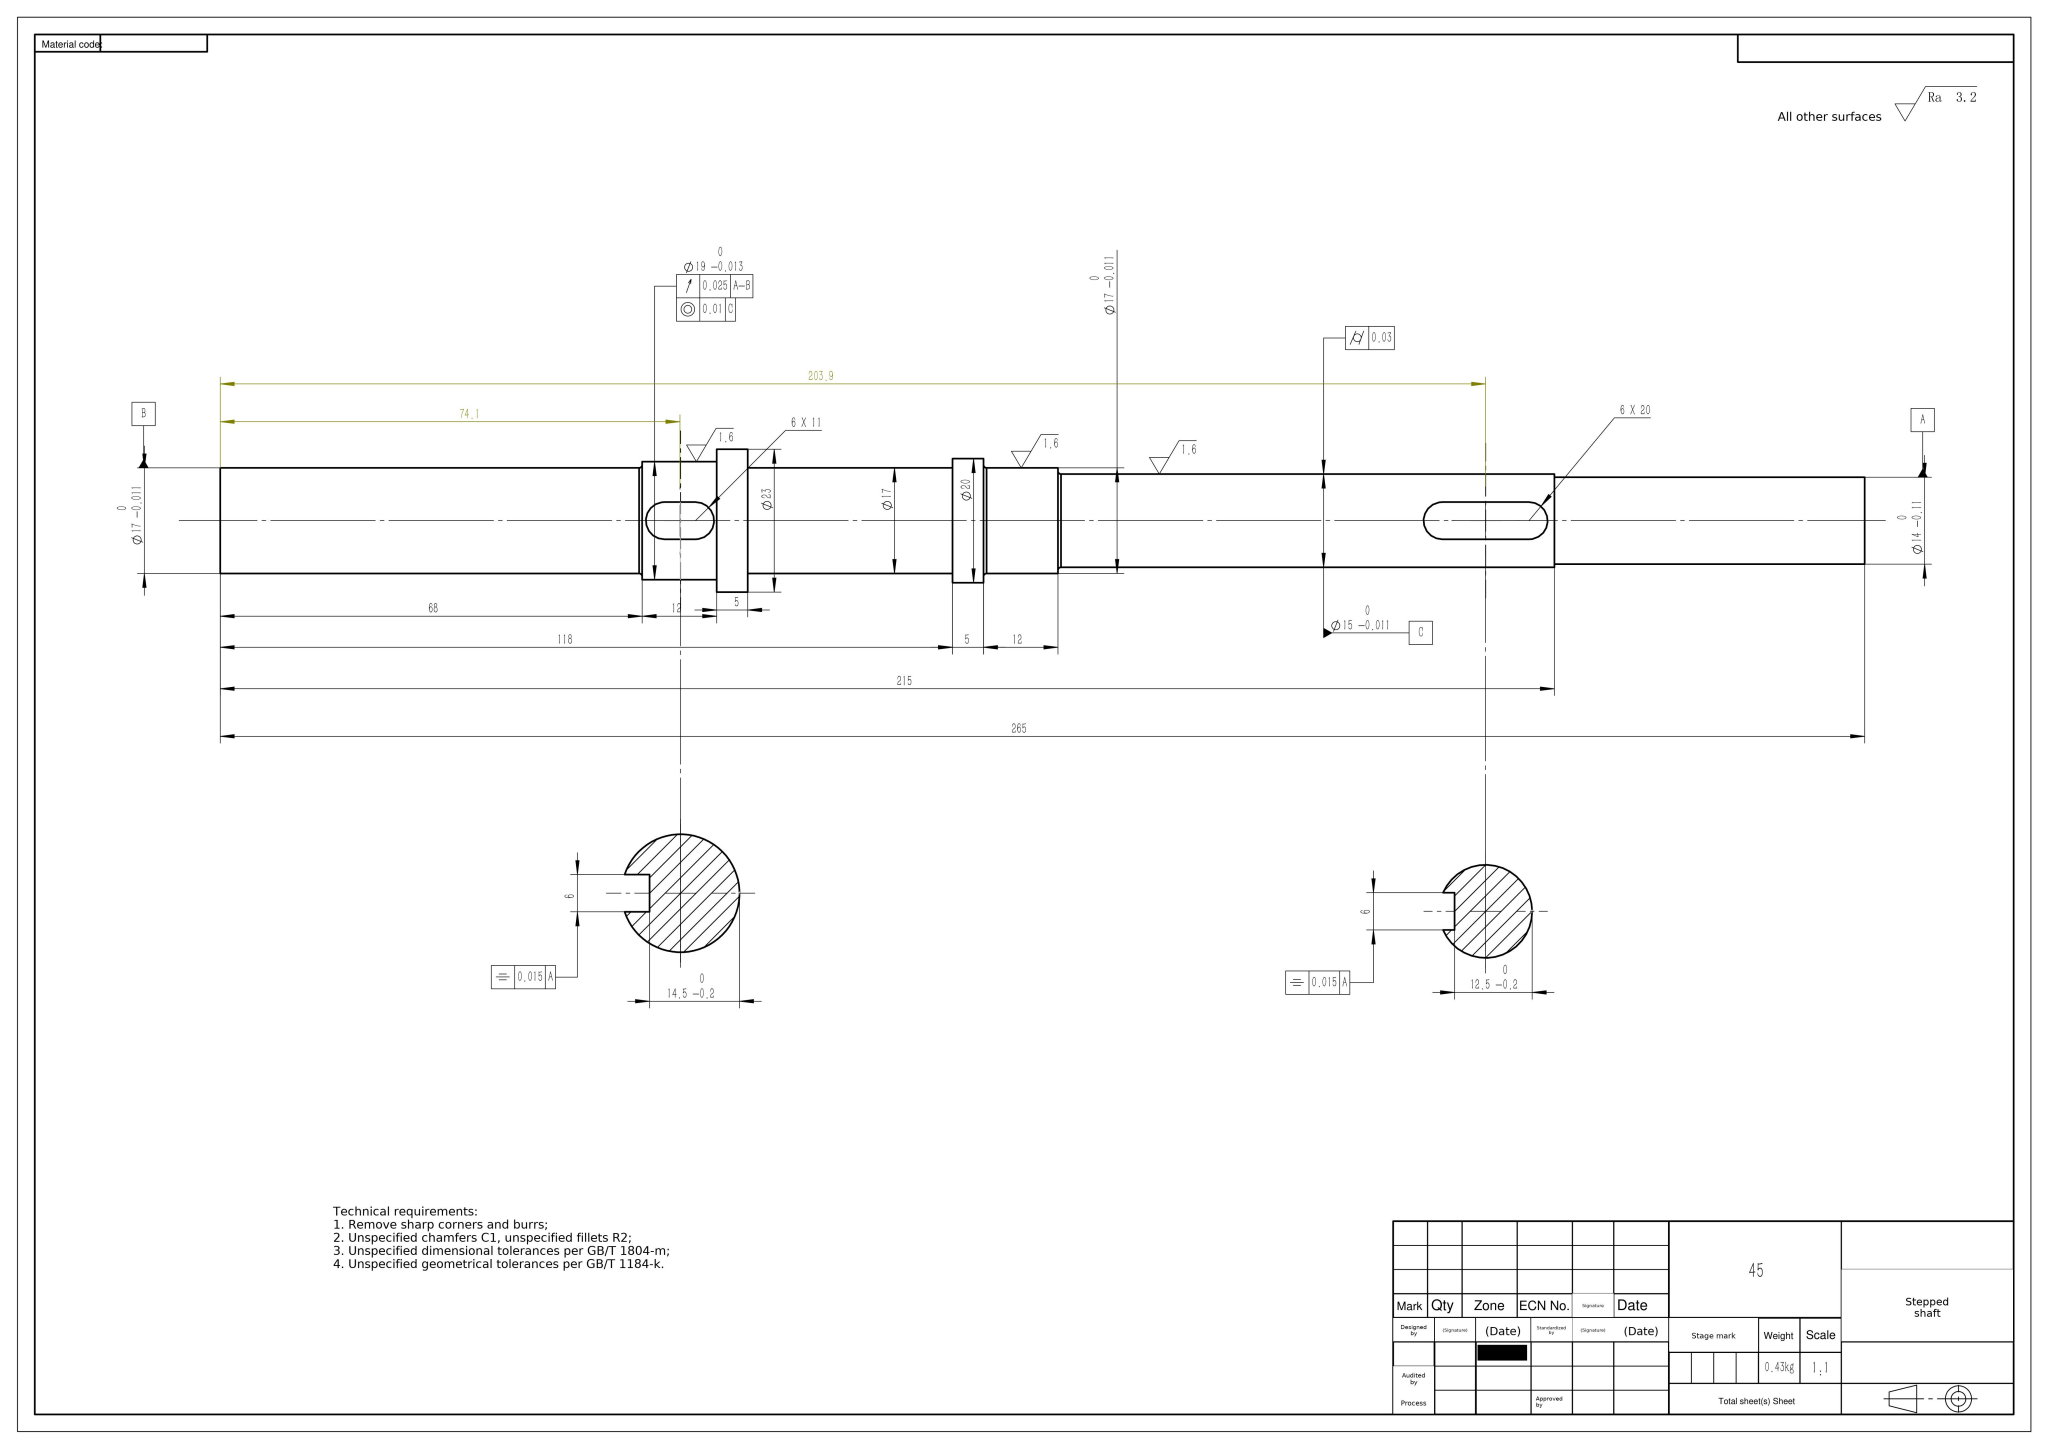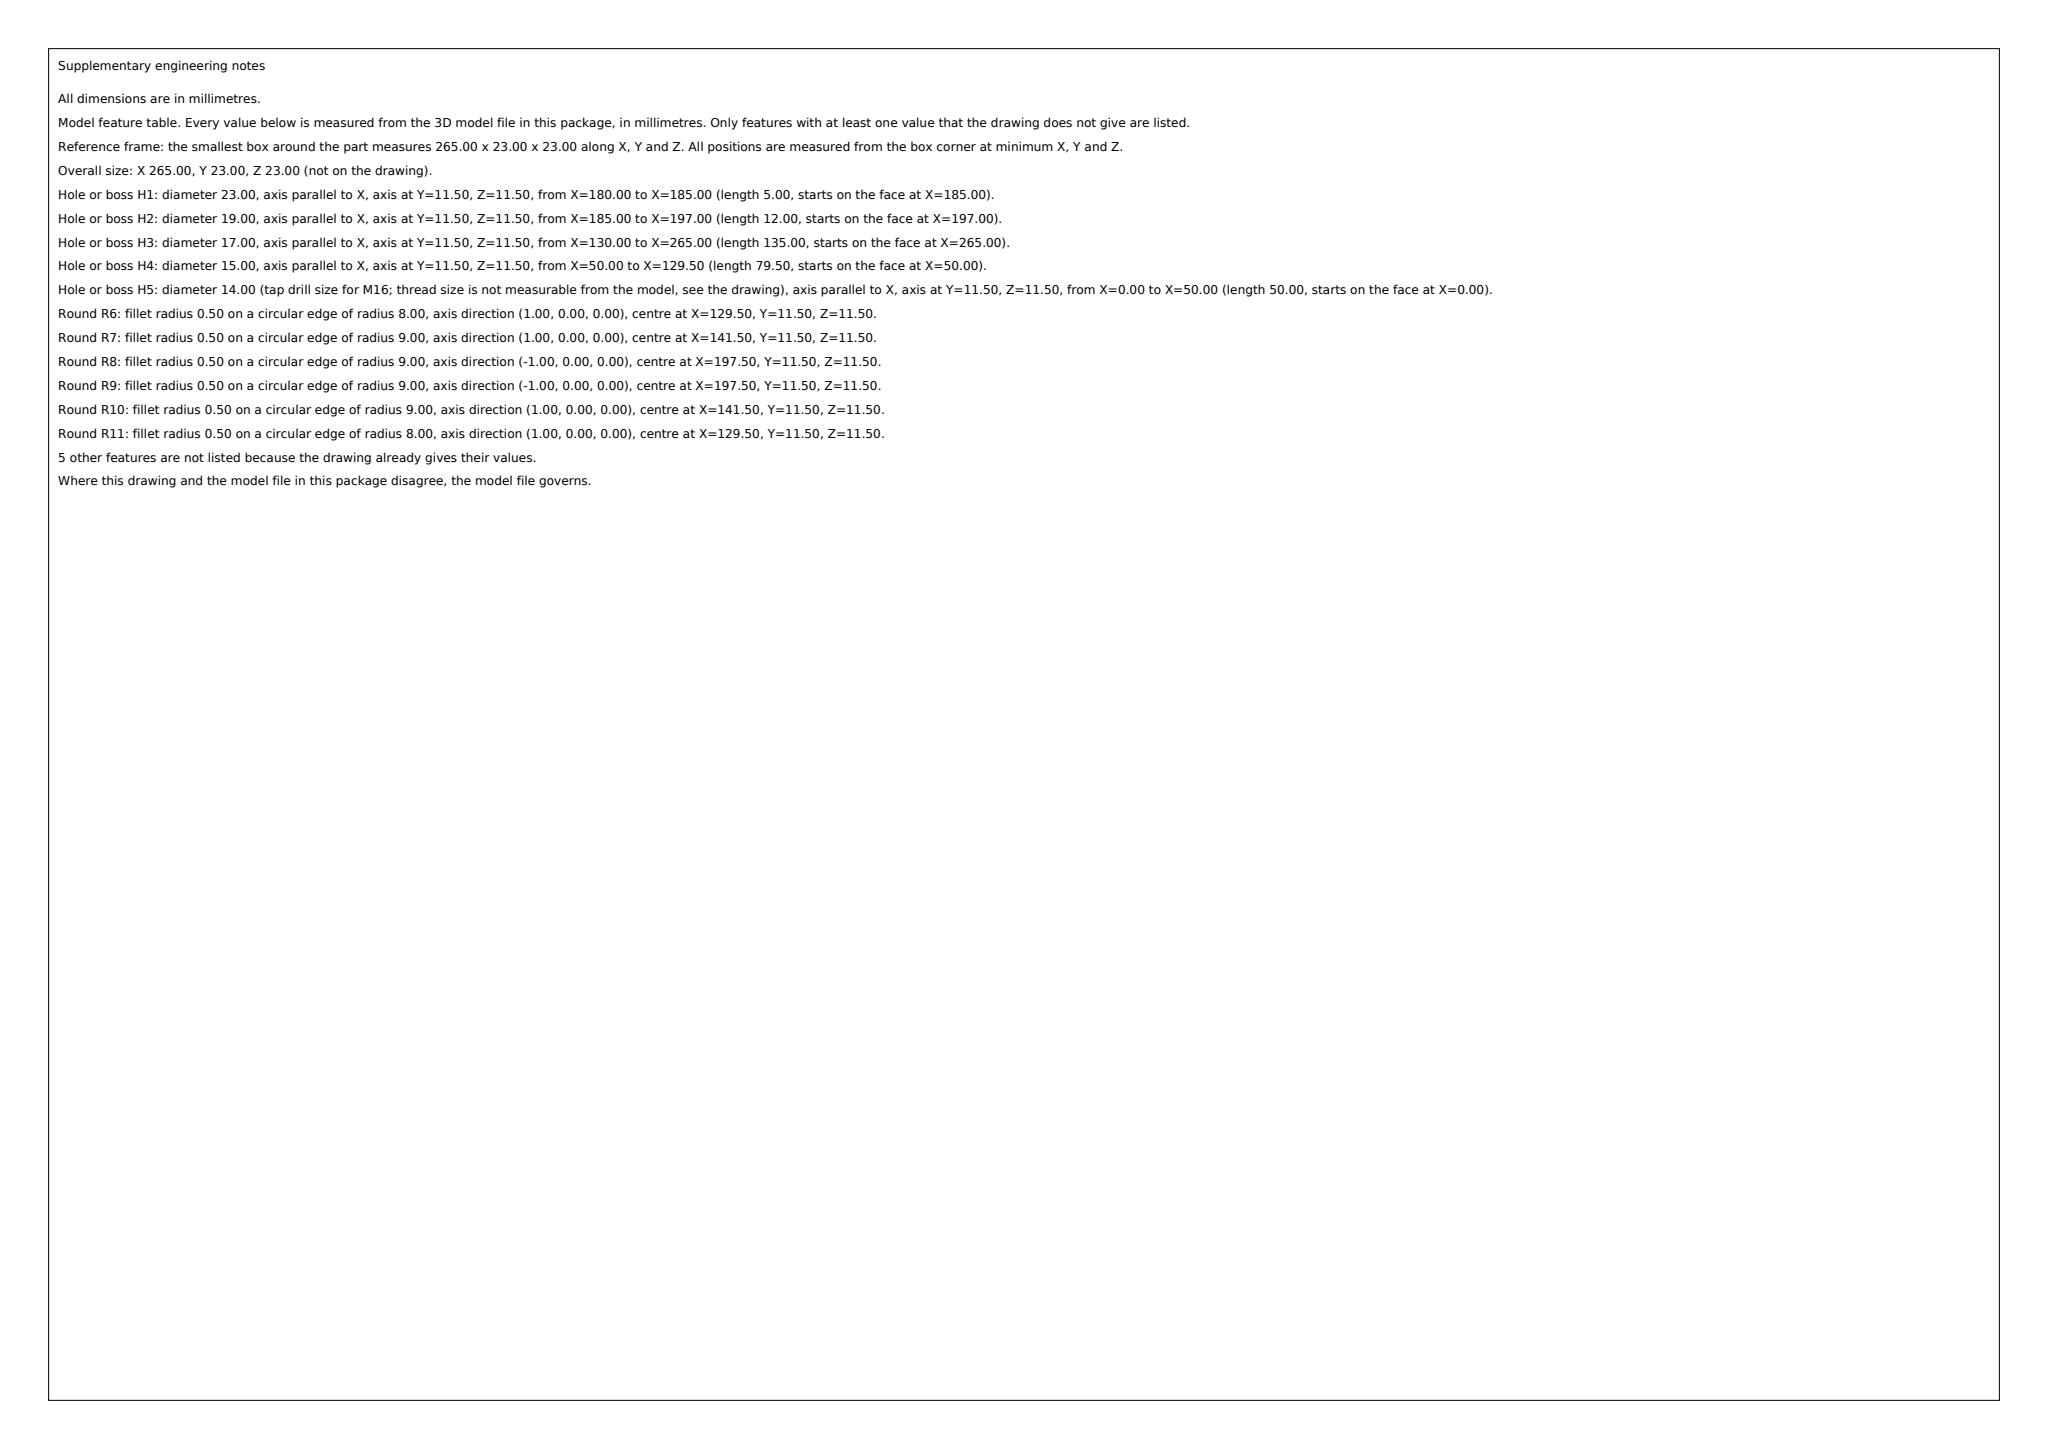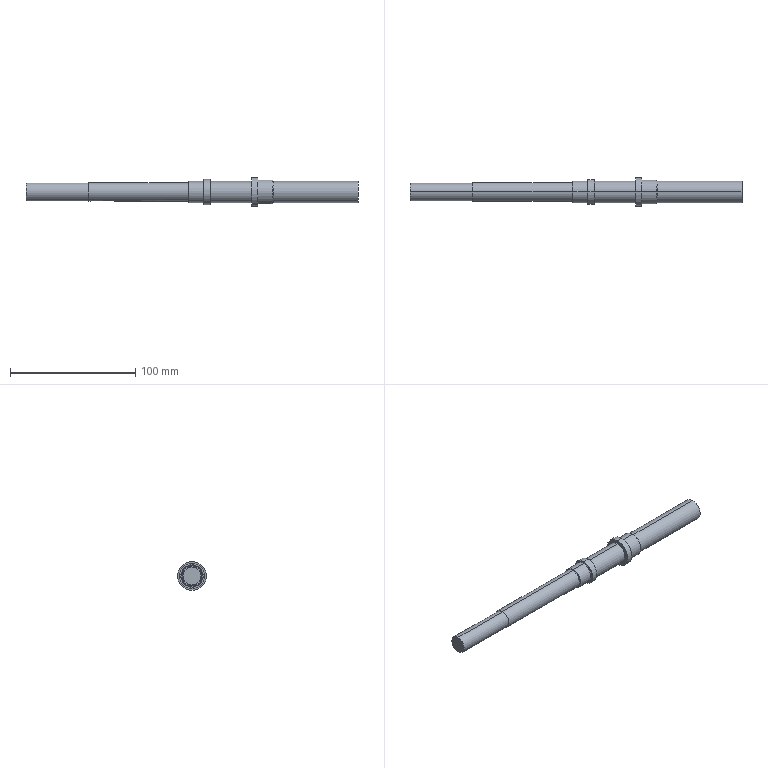Part | SolidWorks | mm | 1 solid | 43 faces | box 265 x 23 x 23 mm | volume 54029 mm3 | cylinder 22 | plane 15 | torus 6 | commonest cylinder face diameters 6 x6 17 x6 14 x2 19 x2 23 x2 20 x2 15 x2
build123d program:
from build123d import *

# Parameters (mm, degrees)
FILLET1_R           = 0.5
CUT_EXTRUDE2_DEPTH  = 10
CUT_EXTRUDE3_DEPTH  = 10
SKETCH6_R           = 40.607
CUT_EXTRUDE4_DEPTH  = 55
SKETCH7_R           = 7
BOSS_EXTRUDE3_DEPTH = 50


with BuildPart() as part:
    # Sketch1 → Revolve1 (revolve)
    with BuildSketch(Plane.XY, mode=Mode.PRIVATE) as revolve1_sk:
        Polygon((0, 0), (0, 7.5), (80, 7.5), (80, 8.5), (92, 8.5), (92, 10), (97, 10), (97, 8.5), (130, 8.5), (130, 11.5), (135, 11.5), (135, 9.5), (147, 9.5), (147, 8.5), (250, 8.5), (250, 7.191), (270, 7.191), (270, 0), align=None)
    revolve(revolve1_sk.sketch.rotate(Axis((0, 0, 0), (1, 0, 0)), 90), axis=Axis((0, 0, 0), (1, 0, 0)))

    # Fillet1
    fillet1_edges = [part.edges().sort_by_distance(p)[0] for p in [
        (250, 0, -7.191),
        (147, 0, -8.5),
        (92, 0, -8.5),
        (80, 0, -7.5),
    ]]
    fillet(fillet1_edges, radius=FILLET1_R)

    # Sketch3 → Cut-Extrude2 (cut)
    with BuildSketch(Plane.XY.offset(-5)):
        with BuildLine():
            Line((4.086, 3), (18.086, 3))
            ThreePointArc((18.086, 3), (21.086, 0), (18.086, -3))
            Line((18.086, -3), (4.086, -3))
            ThreePointArc((4.086, -3), (1.086, 0), (4.086, 3))
        make_face()
    extrude(amount=-CUT_EXTRUDE2_DEPTH, mode=Mode.SUBTRACT)

    # Sketch4 → Cut-Extrude3 (cut)
    with BuildSketch(Plane.XY.offset(-5)):
        with BuildLine():
            Line((138.414, 3), (143.414, 3))
            ThreePointArc((143.414, 3), (146.414, 0), (143.414, -3))
            Line((143.414, -3), (138.414, -3))
            ThreePointArc((138.414, -3), (135.414, 0), (138.414, 3))
        make_face()
    extrude(amount=-CUT_EXTRUDE3_DEPTH, mode=Mode.SUBTRACT)

    # Sketch6 → Cut-Extrude4 (cut)
    with BuildSketch(Plane(origin=(270, 0, 0), x_dir=(0, 0, -1), z_dir=(1, 0, 0))):
        Circle(SKETCH6_R)
    extrude(amount=-CUT_EXTRUDE4_DEPTH, mode=Mode.SUBTRACT)

    # Sketch7 → Boss-Extrude3 (add)
    with BuildSketch(Plane.ZY):
        with Locations(Location((0, 0, 0), (0, 0, 180))):
            Circle(SKETCH7_R)
    extrude(amount=BOSS_EXTRUDE3_DEPTH)


solid = part.part